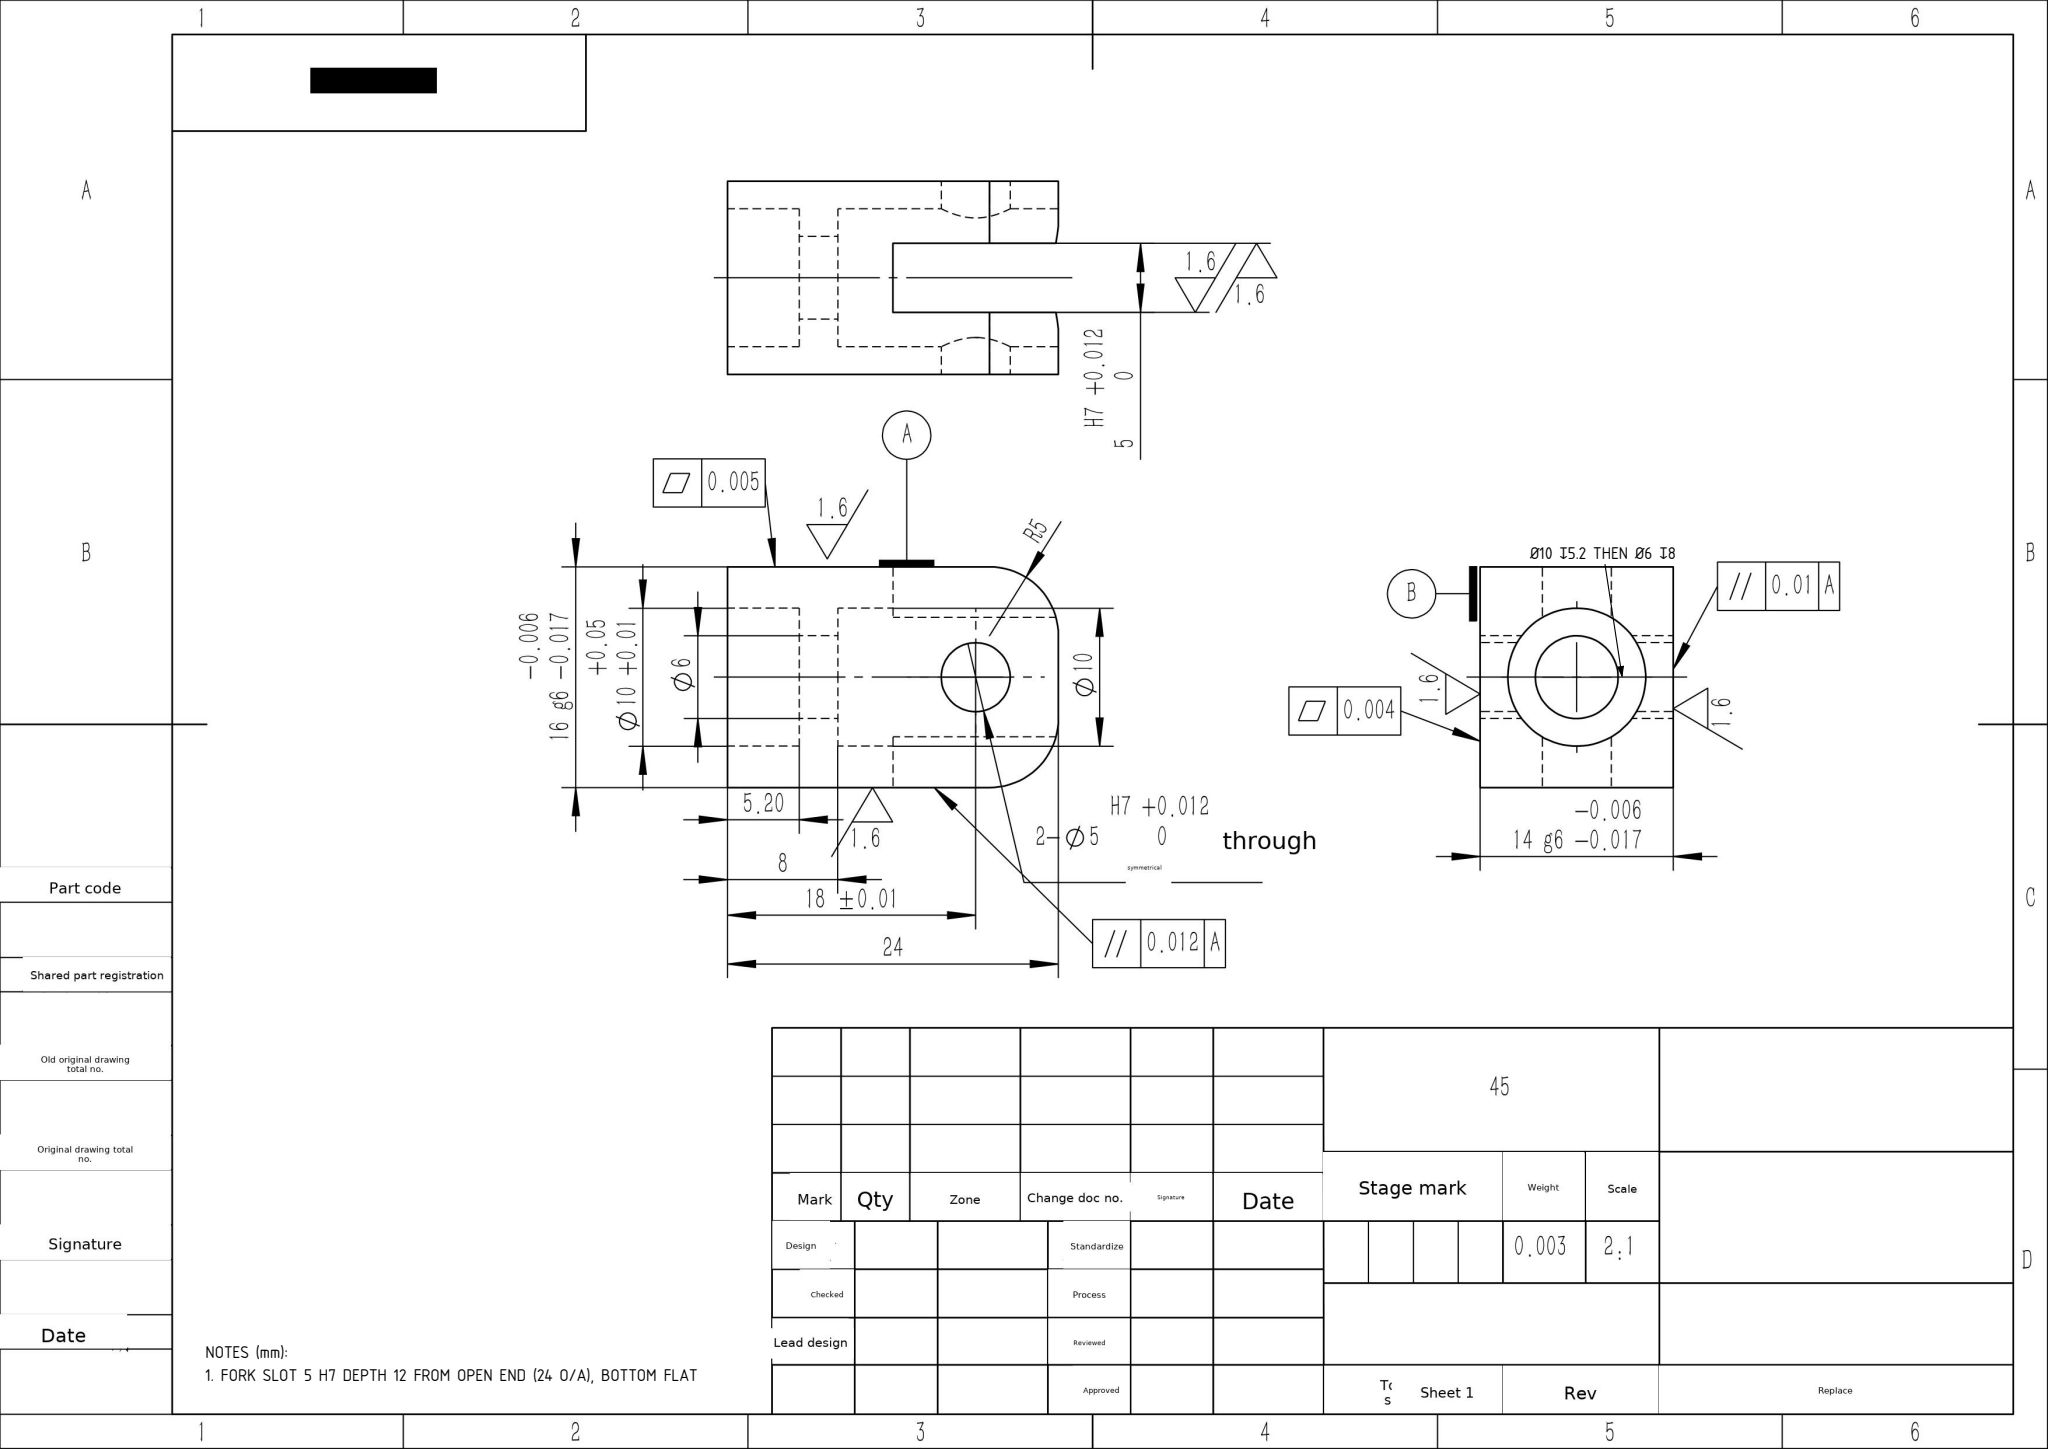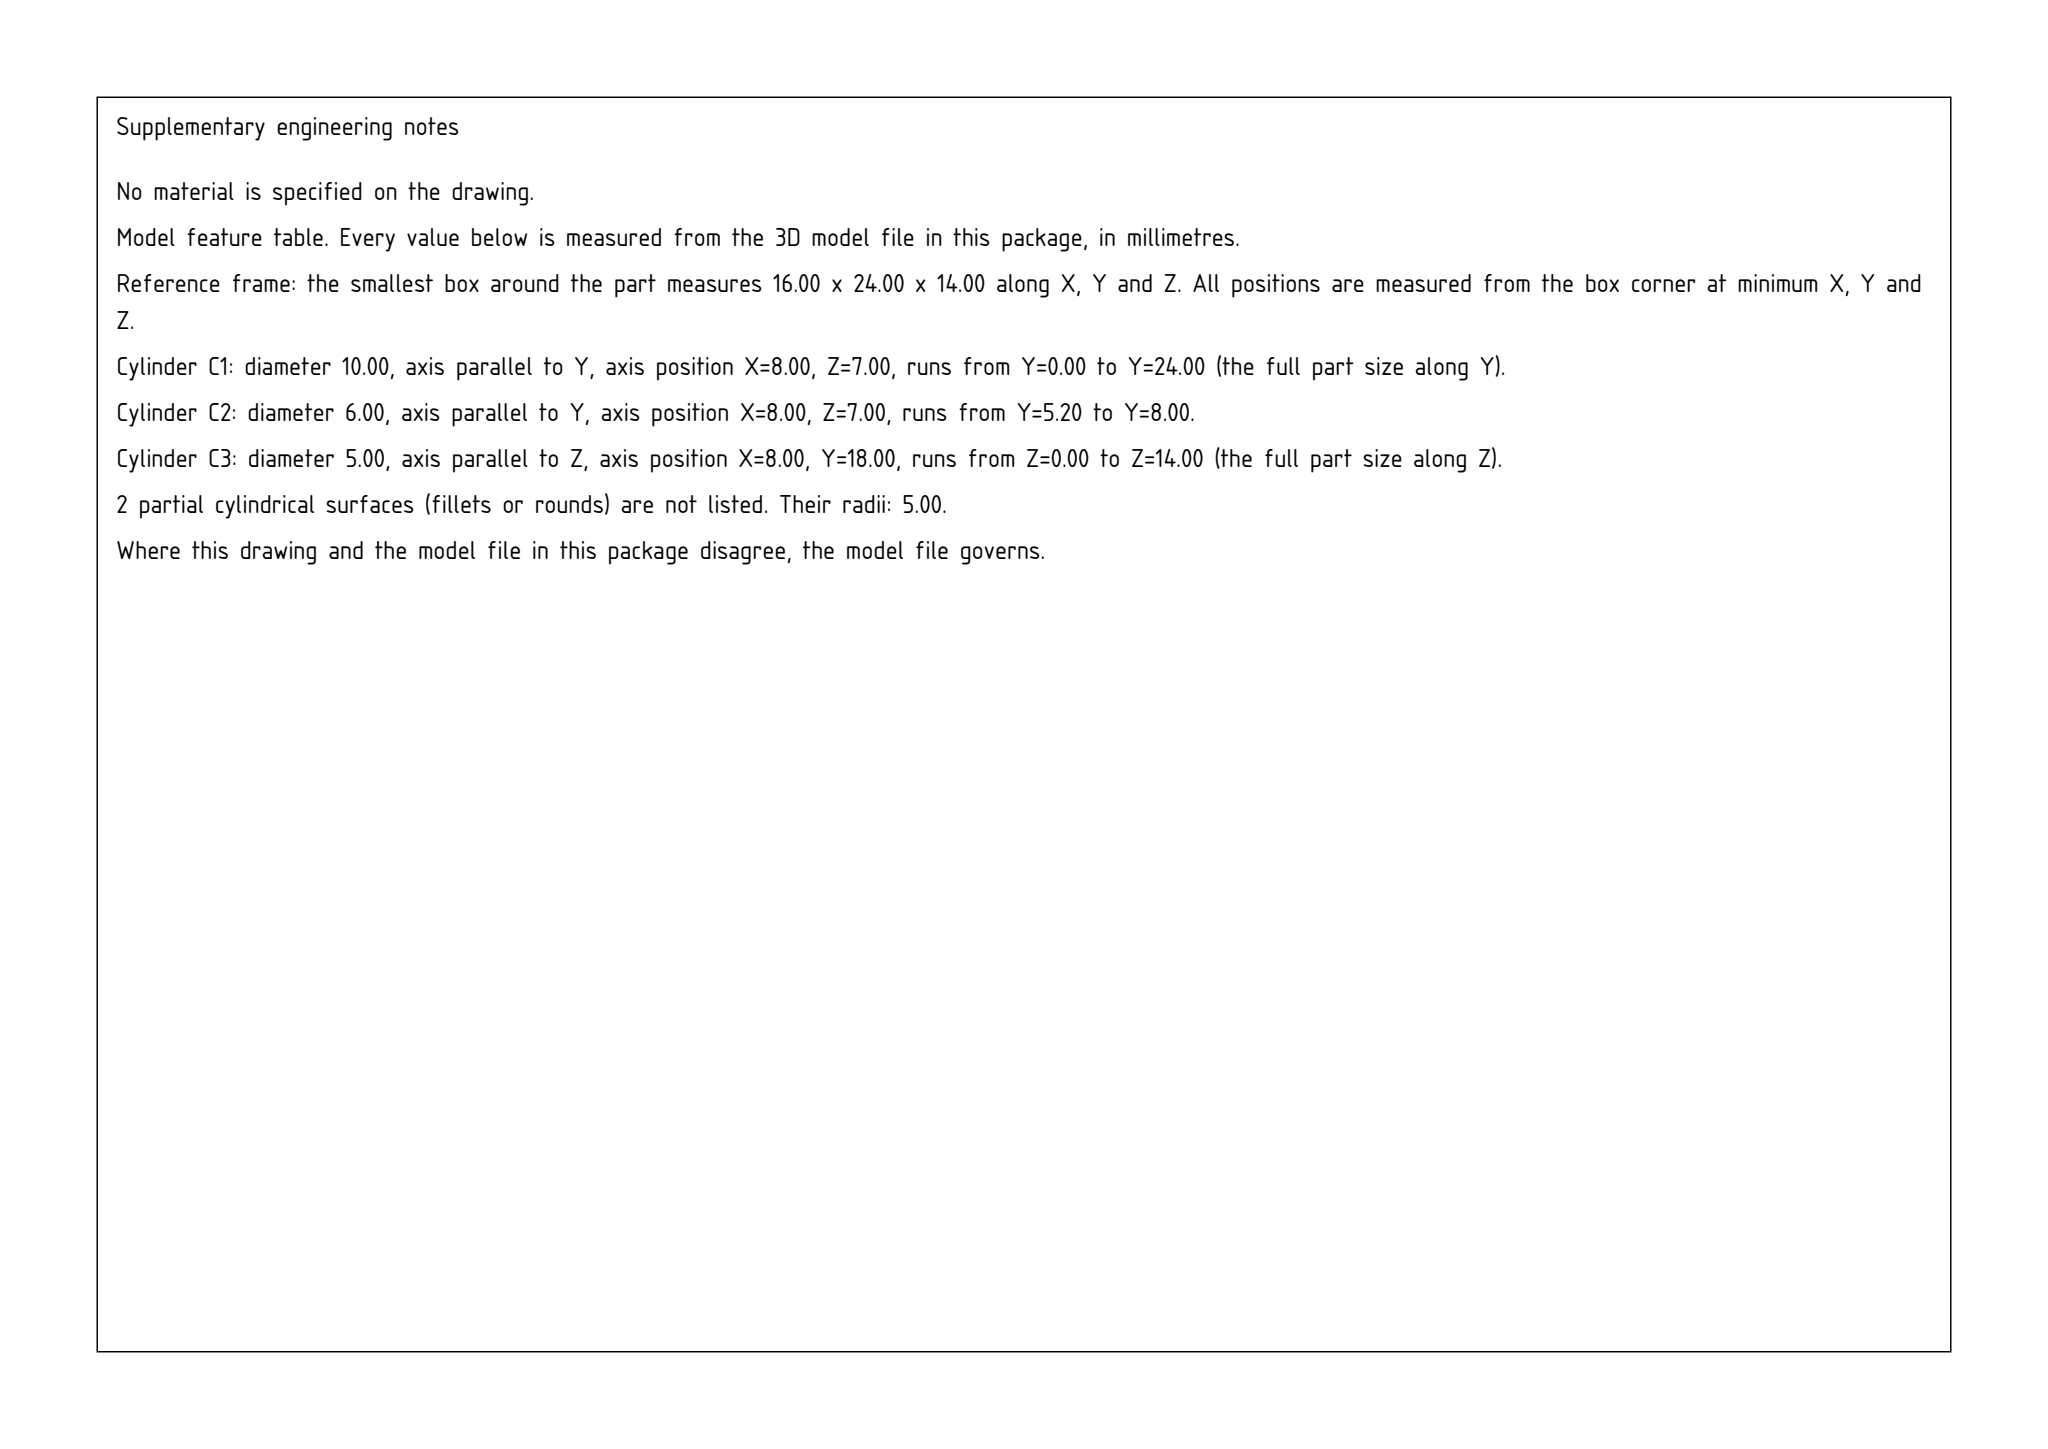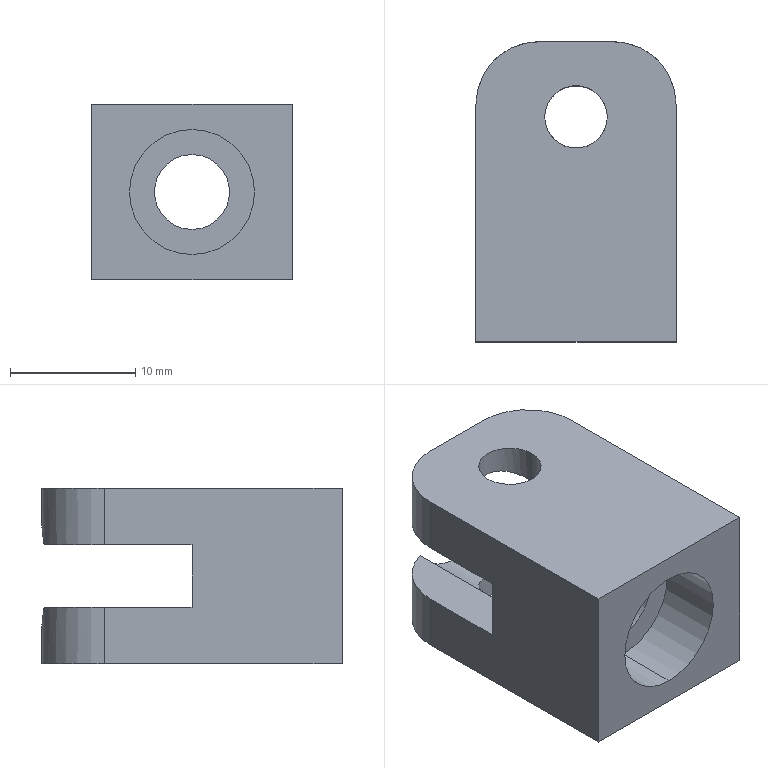Part | SolidWorks | mm | material 45 | 1 solid | 29 faces | box 16 x 24 x 14 mm | volume 3064 mm3 | plane 15 | cylinder 14 | commonest cylinder face diameters 10 x8 5 x4 6 x2
Drawing notes:
FORK SLOT 5 H7 DEPTH 12 FROM OPEN END (24 O/A), BOTTOM FLAT | from the solid: y-planes at 12.0 (2) and 24.0 (2); bbox Y=24 -> slot bottom 12 from end face
Ø10 BORE HT 5.2 FROM END FACE, THEN Ø6 TO 8 DEEP | from the solid: Ø10 bore axis y, from 0.0 to 5.2; Ø6 bore from 5.2 to 8.0 (same axis at x8,z7)
build123d program:
from build123d import *

# Parameters (mm, degrees)
SKETCH1_W           = 16
SKETCH1_H           = 24
BOSS_EXTRUDE1_DEPTH = 14
SKETCH2_R           = 5
CUT_EXTRUDE1_DEPTH  = 16
SKETCH3_W           = 43.143
SKETCH3_H           = 5
CUT_EXTRUDE2_DEPTH  = 12
SKETCH4_R           = 3
CUT_EXTRUDE3_DEPTH  = 27.608
CUT_EXTRUDE4_START  = -5.2
SKETCH5_R           = 5
CUT_EXTRUDE4_DEPTH  = 5.2
SKETCH6_R           = 2.5
CUT_EXTRUDE5_DEPTH  = 33.062
FILLET1_R           = 5


with BuildPart() as part:
    # Sketch1 → Boss-Extrude1 (new body)
    with BuildSketch(Plane.XY):
        with Locations((8, 12)):
            Rectangle(SKETCH1_W, SKETCH1_H)
    extrude(amount=BOSS_EXTRUDE1_DEPTH)

    # Sketch2 → Cut-Extrude1 (cut)
    with BuildSketch(Plane(origin=(0, 24, 0), x_dir=(1, 0, 0), z_dir=(0, 1, 0))):
        with Locations(Location((8, -7, 0), (0, 0, 270))):
            Circle(SKETCH2_R)
    extrude(amount=-CUT_EXTRUDE1_DEPTH, mode=Mode.SUBTRACT)

    # Sketch3 → Cut-Extrude2 (cut)
    with BuildSketch(Plane(origin=(0, 24, 0), x_dir=(1, 0, 0), z_dir=(0, 1, 0))):
        with Locations((0, -7)):
            Rectangle(SKETCH3_W, SKETCH3_H)
    extrude(amount=-CUT_EXTRUDE2_DEPTH, mode=Mode.SUBTRACT)

    # Sketch4 → Cut-Extrude3 (cut, through all)
    with BuildSketch(Plane(origin=(0, 8, 0), x_dir=(1, 0, 0), z_dir=(0, 1, 0))):
        with Locations(Location((8, -7, 0), (0, 0, 270))):
            Circle(SKETCH4_R)
    extrude(amount=-CUT_EXTRUDE3_DEPTH, mode=Mode.SUBTRACT)

    # Sketch5 → Cut-Extrude4 (cut)
    with BuildSketch(Plane.XZ.offset(CUT_EXTRUDE4_START)):
        with Locations(Location((8, 7, 0), (0, 0, 90))):
            Circle(SKETCH5_R)
    extrude(amount=CUT_EXTRUDE4_DEPTH, mode=Mode.SUBTRACT)

    # Sketch6 → Cut-Extrude5 (cut, through all)
    with BuildSketch(Plane.XY.offset(14)):
        with Locations((8, 18)):
            Circle(SKETCH6_R)
    extrude(amount=-CUT_EXTRUDE5_DEPTH, mode=Mode.SUBTRACT)

    # Fillet1
    fillet1_edges = [part.edges().sort_by_distance(p)[0] for p in [
        (0, 24, 2.25),
        (16, 24, 2.25),
        (16, 24, 11.75),
        (0, 24, 11.75),
    ]]
    fillet(fillet1_edges, radius=FILLET1_R)


solid = part.part